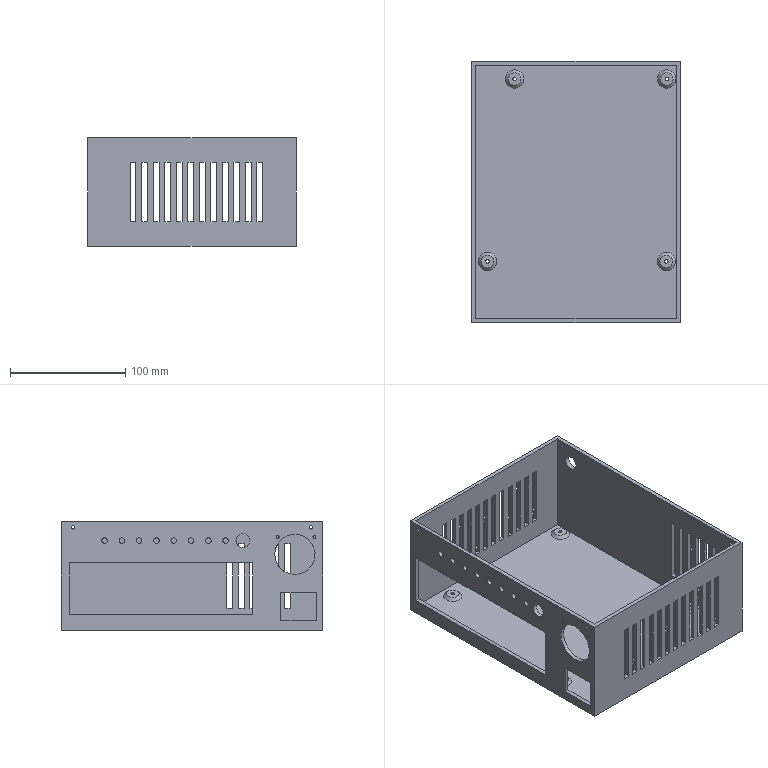Component | NX | WAIKE | 1 solid | 196 faces | volume 339307 mm3 | plane 171 | cylinder 21 | cone 4 | commonest cylinder face diameters 3 x8 4.85 x8 2.61 x2 12 x2 35 x1